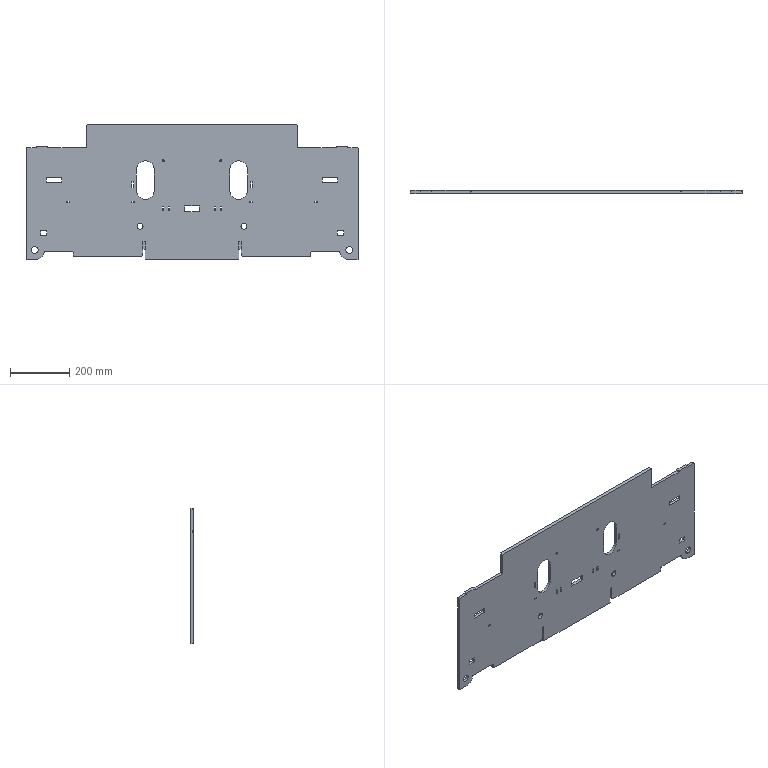Component | SolidWorks | FrontUprightPlate-1 | 1 solid | 141 faces | volume 4496478 mm3 | plane 107 | cylinder 34 | commonest cylinder face diameters 5.2 x8 20.2 x4 7.2 x4 23.2 x4 10 x4 60 x4 20 x2 6 x2 | material Q235